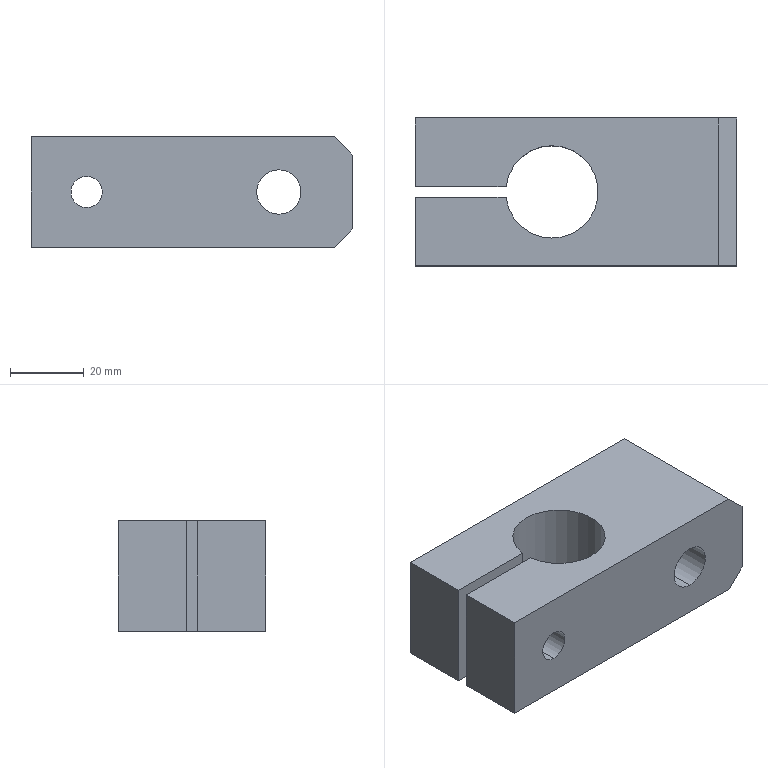Component | SolidWorks | DirectPressureVerticalSeal-1_VerticalSealMainArmFixingFrame-1 | 1 solid | 20 faces | box 87 x 40 x 30 mm | volume 79126 mm3 | plane 11 | cylinder 7 | cone 2 | commonest cylinder face diameters 11 x2 12 x2 8.5 x2 25 x1
STEP:
#1=CARTESIAN_POINT('',(-20.502,9.63,11.191));
#2=VERTEX_POINT('',#1);
#3=CARTESIAN_POINT('',(-20.502,9.63,11.526));
#4=VERTEX_POINT('',#3);
#5=CARTESIAN_POINT('',(-20.502,9.63,11.358));
#6=DIRECTION('',(0.,1.,0.));
#7=DIRECTION('',(0.,0.,-1.));
#8=AXIS2_PLACEMENT_3D('',#5,#6,#7);
#9=CIRCLE('',#8,0.1673);
#10=EDGE_CURVE('',#2,#4,#9,.T.);
#11=ORIENTED_EDGE('',*,*,#10,.F.);
#12=CARTESIAN_POINT('',(-20.502,9.66,11.16));
#13=VERTEX_POINT('',#12);
#14=CARTESIAN_POINT('',(-20.502,9.63,11.191));
#15=DIRECTION('',(0.,0.7071,-0.7071));
#16=VECTOR('',#15,39.37);
#17=LINE('',#14,#16);
#18=EDGE_CURVE('',#2,#13,#17,.T.);
#19=ORIENTED_EDGE('',*,*,#18,.T.);
#20=CARTESIAN_POINT('',(-20.502,9.66,11.556));
#21=VERTEX_POINT('',#20);
#22=CARTESIAN_POINT('',(-20.502,9.66,11.358));
#23=DIRECTION('',(-0.,-1.,0.));
#24=DIRECTION('',(1.,0.,0.));
#25=AXIS2_PLACEMENT_3D('',#22,#23,#24);
#26=CIRCLE('',#25,0.1978);
#27=EDGE_CURVE('',#21,#13,#26,.T.);
#28=ORIENTED_EDGE('',*,*,#27,.F.);
#29=CARTESIAN_POINT('',(-20.502,9.63,11.526));
#30=DIRECTION('',(0.,0.7071,0.7071));
#31=VECTOR('',#30,39.37);
#32=LINE('',#29,#31);
#33=EDGE_CURVE('',#4,#21,#32,.T.);
#34=ORIENTED_EDGE('',*,*,#33,.F.);
#35=EDGE_LOOP('',(#11,#19,#28,#34));
#36=FACE_OUTER_BOUND('',#35,.T.);
#37=CARTESIAN_POINT('',(-20.502,9.63,11.358));
#38=DIRECTION('',(0.,1.,0.));
#39=DIRECTION('',(0.,0.,1.));
#40=AXIS2_PLACEMENT_3D('',#37,#38,#39);
#41=CONICAL_SURFACE('',#40,0.1673,0.7854);
#42=ADVANCED_FACE('',(#36),#41,.F.);
#43=CARTESIAN_POINT('',(-20.502,10.507,11.575));
#44=VERTEX_POINT('',#43);
#45=CARTESIAN_POINT('',(-20.502,10.507,11.142));
#46=VERTEX_POINT('',#45);
#47=CARTESIAN_POINT('',(-20.502,10.507,11.358));
#48=DIRECTION('',(0.,-1.,0.));
#49=DIRECTION('',(0.,0.,-1.));
#50=AXIS2_PLACEMENT_3D('',#47,#48,#49);
#51=CIRCLE('',#50,0.2165);
#52=EDGE_CURVE('',#44,#46,#51,.T.);
#53=ORIENTED_EDGE('',*,*,#52,.F.);
#54=CARTESIAN_POINT('',(-20.502,9.778,11.575));
#55=VERTEX_POINT('',#54);
#56=CARTESIAN_POINT('',(-20.502,9.778,11.575));
#57=DIRECTION('',(0.,-1.,0.));
#58=VECTOR('',#57,39.37);
#59=LINE('',#56,#58);
#60=EDGE_CURVE('',#44,#55,#59,.T.);
#61=ORIENTED_EDGE('',*,*,#60,.T.);
#62=CARTESIAN_POINT('',(-20.502,9.778,11.142));
#63=VERTEX_POINT('',#62);
#64=CARTESIAN_POINT('',(-20.502,9.778,11.358));
#65=DIRECTION('',(0.,-1.,0.));
#66=DIRECTION('',(0.,0.,-1.));
#67=AXIS2_PLACEMENT_3D('',#64,#65,#66);
#68=CIRCLE('',#67,0.2165);
#69=EDGE_CURVE('',#55,#63,#68,.T.);
#70=ORIENTED_EDGE('',*,*,#69,.T.);
#71=CARTESIAN_POINT('',(-20.502,9.778,11.142));
#72=DIRECTION('',(0.,-1.,0.));
#73=VECTOR('',#72,39.37);
#74=LINE('',#71,#73);
#75=EDGE_CURVE('',#46,#63,#74,.T.);
#76=ORIENTED_EDGE('',*,*,#75,.F.);
#77=EDGE_LOOP('',(#53,#61,#70,#76));
#78=FACE_OUTER_BOUND('',#77,.T.);
#79=CARTESIAN_POINT('',(-20.502,9.778,11.358));
#80=DIRECTION('',(0.,-1.,0.));
#81=DIRECTION('',(0.,0.,-1.));
#82=AXIS2_PLACEMENT_3D('',#79,#80,#81);
#83=CYLINDRICAL_SURFACE('',#82,0.2165);
#84=ADVANCED_FACE('',(#78),#83,.F.);
#85=CARTESIAN_POINT('',(-18.455,10.507,11.594));
#86=VERTEX_POINT('',#85);
#87=CARTESIAN_POINT('',(-18.455,10.507,11.122));
#88=VERTEX_POINT('',#87);
#89=CARTESIAN_POINT('',(-18.455,10.507,11.358));
#90=DIRECTION('',(0.,-1.,0.));
#91=DIRECTION('',(0.,0.,-1.));
#92=AXIS2_PLACEMENT_3D('',#89,#90,#91);
#93=CIRCLE('',#92,0.2362);
#94=EDGE_CURVE('',#86,#88,#93,.T.);
#95=ORIENTED_EDGE('',*,*,#94,.F.);
#96=CARTESIAN_POINT('',(-18.455,8.932,11.594));
#97=VERTEX_POINT('',#96);
#98=CARTESIAN_POINT('',(-18.455,8.932,11.594));
#99=DIRECTION('',(0.,-1.,0.));
#100=VECTOR('',#99,39.37);
#101=LINE('',#98,#100);
#102=EDGE_CURVE('',#86,#97,#101,.T.);
#103=ORIENTED_EDGE('',*,*,#102,.T.);
#104=CARTESIAN_POINT('',(-18.455,8.932,11.122));
#105=VERTEX_POINT('',#104);
#106=CARTESIAN_POINT('',(-18.455,8.932,11.358));
#107=DIRECTION('',(0.,-1.,0.));
#108=DIRECTION('',(0.,0.,-1.));
#109=AXIS2_PLACEMENT_3D('',#106,#107,#108);
#110=CIRCLE('',#109,0.2362);
#111=EDGE_CURVE('',#97,#105,#110,.T.);
#112=ORIENTED_EDGE('',*,*,#111,.T.);
#113=CARTESIAN_POINT('',(-18.455,8.932,11.122));
#114=DIRECTION('',(0.,-1.,0.));
#115=VECTOR('',#114,39.37);
#116=LINE('',#113,#115);
#117=EDGE_CURVE('',#88,#105,#116,.T.);
#118=ORIENTED_EDGE('',*,*,#117,.F.);
#119=EDGE_LOOP('',(#95,#103,#112,#118));
#120=FACE_OUTER_BOUND('',#119,.T.);
#121=CARTESIAN_POINT('',(-18.455,8.932,11.358));
#122=DIRECTION('',(0.,-1.,0.));
#123=DIRECTION('',(0.,0.,-1.));
#124=AXIS2_PLACEMENT_3D('',#121,#122,#123);
#125=CYLINDRICAL_SURFACE('',#124,0.2362);
#126=ADVANCED_FACE('',(#120),#125,.F.);
#127=CARTESIAN_POINT('',(-20.502,8.932,11.191));
#128=VERTEX_POINT('',#127);
#129=CARTESIAN_POINT('',(-20.502,8.932,11.526));
#130=VERTEX_POINT('',#129);
#131=CARTESIAN_POINT('',(-20.502,8.932,11.358));
#132=DIRECTION('',(0.,1.,0.));
#133=DIRECTION('',(0.,0.,1.));
#134=AXIS2_PLACEMENT_3D('',#131,#132,#133);
#135=CIRCLE('',#134,0.1673);
#136=EDGE_CURVE('',#128,#130,#135,.T.);
#137=ORIENTED_EDGE('',*,*,#136,.F.);
#138=CARTESIAN_POINT('',(-20.502,9.66,11.191));
#139=DIRECTION('',(0.,1.,0.));
#140=VECTOR('',#139,39.37);
#141=LINE('',#138,#140);
#142=EDGE_CURVE('',#128,#2,#141,.T.);
#143=ORIENTED_EDGE('',*,*,#142,.T.);
#144=ORIENTED_EDGE('',*,*,#10,.T.);
#145=CARTESIAN_POINT('',(-20.502,9.66,11.526));
#146=DIRECTION('',(0.,1.,0.));
#147=VECTOR('',#146,39.37);
#148=LINE('',#145,#147);
#149=EDGE_CURVE('',#130,#4,#148,.T.);
#150=ORIENTED_EDGE('',*,*,#149,.F.);
#151=EDGE_LOOP('',(#137,#143,#144,#150));
#152=FACE_OUTER_BOUND('',#151,.T.);
#153=CARTESIAN_POINT('',(-20.502,9.66,11.358));
#154=DIRECTION('',(0.,1.,0.));
#155=DIRECTION('',(0.,0.,1.));
#156=AXIS2_PLACEMENT_3D('',#153,#154,#155);
#157=CYLINDRICAL_SURFACE('',#156,0.1673);
#158=ADVANCED_FACE('',(#152),#157,.F.);
#159=CARTESIAN_POINT('',(-21.092,9.66,11.949));
#160=VERTEX_POINT('',#159);
#161=CARTESIAN_POINT('',(-21.092,9.66,10.768));
#162=VERTEX_POINT('',#161);
#163=CARTESIAN_POINT('',(-21.092,9.66,11.949));
#164=DIRECTION('',(0.,0.,-1.));
#165=VECTOR('',#164,39.37);
#166=LINE('',#163,#165);
#167=EDGE_CURVE('',#160,#162,#166,.T.);
#168=ORIENTED_EDGE('',*,*,#167,.T.);
#169=CARTESIAN_POINT('',(-21.092,8.932,10.768));
#170=VERTEX_POINT('',#169);
#171=CARTESIAN_POINT('',(-21.092,10.507,10.768));
#172=DIRECTION('',(0.,-1.,0.));
#173=VECTOR('',#172,39.37);
#174=LINE('',#171,#173);
#175=EDGE_CURVE('',#162,#170,#174,.T.);
#176=ORIENTED_EDGE('',*,*,#175,.T.);
#177=CARTESIAN_POINT('',(-21.092,8.932,11.949));
#178=VERTEX_POINT('',#177);
#179=CARTESIAN_POINT('',(-21.092,8.932,10.768));
#180=DIRECTION('',(0.,0.,1.));
#181=VECTOR('',#180,39.37);
#182=LINE('',#179,#181);
#183=EDGE_CURVE('',#170,#178,#182,.T.);
#184=ORIENTED_EDGE('',*,*,#183,.T.);
#185=CARTESIAN_POINT('',(-21.092,10.507,11.949));
#186=DIRECTION('',(0.,-1.,0.));
#187=VECTOR('',#186,39.37);
#188=LINE('',#185,#187);
#189=EDGE_CURVE('',#160,#178,#188,.T.);
#190=ORIENTED_EDGE('',*,*,#189,.F.);
#191=EDGE_LOOP('',(#168,#176,#184,#190));
#192=FACE_OUTER_BOUND('',#191,.T.);
#193=CARTESIAN_POINT('',(-21.092,10.507,10.768));
#194=DIRECTION('',(-1.,0.,0.));
#195=DIRECTION('',(0.,0.,1.));
#196=AXIS2_PLACEMENT_3D('',#193,#194,#195);
#197=PLANE('',#196);
#198=ADVANCED_FACE('',(#192),#197,.T.);
#199=CARTESIAN_POINT('',(-17.667,8.932,10.965));
#200=VERTEX_POINT('',#199);
#201=CARTESIAN_POINT('',(-17.667,8.932,11.752));
#202=VERTEX_POINT('',#201);
#203=CARTESIAN_POINT('',(-17.667,8.932,10.768));
#204=DIRECTION('',(0.,0.,1.));
#205=VECTOR('',#204,39.37);
#206=LINE('',#203,#205);
#207=EDGE_CURVE('',#200,#202,#206,.T.);
#208=ORIENTED_EDGE('',*,*,#207,.F.);
#209=CARTESIAN_POINT('',(-17.667,10.507,10.965));
#210=VERTEX_POINT('',#209);
#211=CARTESIAN_POINT('',(-17.667,10.507,10.965));
#212=DIRECTION('',(0.,1.,0.));
#213=VECTOR('',#212,39.37);
#214=LINE('',#211,#213);
#215=EDGE_CURVE('',#200,#210,#214,.T.);
#216=ORIENTED_EDGE('',*,*,#215,.T.);
#217=CARTESIAN_POINT('',(-17.667,10.507,11.752));
#218=VERTEX_POINT('',#217);
#219=CARTESIAN_POINT('',(-17.667,10.507,10.768));
#220=DIRECTION('',(0.,0.,1.));
#221=VECTOR('',#220,39.37);
#222=LINE('',#219,#221);
#223=EDGE_CURVE('',#210,#218,#222,.T.);
#224=ORIENTED_EDGE('',*,*,#223,.T.);
#225=CARTESIAN_POINT('',(-17.667,8.932,11.752));
#226=DIRECTION('',(0.,-1.,0.));
#227=VECTOR('',#226,39.37);
#228=LINE('',#225,#227);
#229=EDGE_CURVE('',#218,#202,#228,.T.);
#230=ORIENTED_EDGE('',*,*,#229,.T.);
#231=EDGE_LOOP('',(#208,#216,#224,#230));
#232=FACE_OUTER_BOUND('',#231,.T.);
#233=CARTESIAN_POINT('',(-17.667,8.932,10.768));
#234=DIRECTION('',(1.,0.,0.));
#235=DIRECTION('',(0.,0.,-1.));
#236=AXIS2_PLACEMENT_3D('',#233,#234,#235);
#237=PLANE('',#236);
#238=ADVANCED_FACE('',(#232),#237,.T.);
#239=CARTESIAN_POINT('',(-18.455,8.932,11.358));
#240=DIRECTION('',(0.,-1.,0.));
#241=DIRECTION('',(0.,0.,-1.));
#242=AXIS2_PLACEMENT_3D('',#239,#240,#241);
#243=CIRCLE('',#242,0.2362);
#244=EDGE_CURVE('',#105,#97,#243,.T.);
#245=ORIENTED_EDGE('',*,*,#244,.F.);
#246=ORIENTED_EDGE('',*,*,#111,.F.);
#247=EDGE_LOOP('',(#245,#246));
#248=FACE_BOUND('',#247,.T.);
#249=CARTESIAN_POINT('',(-20.502,8.932,11.358));
#250=DIRECTION('',(0.,1.,0.));
#251=DIRECTION('',(0.,0.,1.));
#252=AXIS2_PLACEMENT_3D('',#249,#250,#251);
#253=CIRCLE('',#252,0.1673);
#254=EDGE_CURVE('',#130,#128,#253,.T.);
#255=ORIENTED_EDGE('',*,*,#254,.T.);
#256=ORIENTED_EDGE('',*,*,#136,.T.);
#257=EDGE_LOOP('',(#255,#256));
#258=FACE_BOUND('',#257,.T.);
#259=CARTESIAN_POINT('',(-17.864,8.932,10.768));
#260=VERTEX_POINT('',#259);
#261=CARTESIAN_POINT('',(-21.092,8.932,10.768));
#262=DIRECTION('',(1.,0.,0.));
#263=VECTOR('',#262,39.37);
#264=LINE('',#261,#263);
#265=EDGE_CURVE('',#170,#260,#264,.T.);
#266=ORIENTED_EDGE('',*,*,#265,.T.);
#267=CARTESIAN_POINT('',(-19.478,8.932,9.154));
#268=DIRECTION('',(0.7071,0.,0.7071));
#269=VECTOR('',#268,39.37);
#270=LINE('',#267,#269);
#271=EDGE_CURVE('',#260,#200,#270,.T.);
#272=ORIENTED_EDGE('',*,*,#271,.T.);
#273=ORIENTED_EDGE('',*,*,#207,.T.);
#274=CARTESIAN_POINT('',(-17.864,8.932,11.949));
#275=VERTEX_POINT('',#274);
#276=CARTESIAN_POINT('',(-18.888,8.932,12.972));
#277=DIRECTION('',(-0.7071,0.,0.7071));
#278=VECTOR('',#277,39.37);
#279=LINE('',#276,#278);
#280=EDGE_CURVE('',#202,#275,#279,.T.);
#281=ORIENTED_EDGE('',*,*,#280,.T.);
#282=CARTESIAN_POINT('',(-21.092,8.932,11.949));
#283=DIRECTION('',(1.,0.,0.));
#284=VECTOR('',#283,39.37);
#285=LINE('',#282,#284);
#286=EDGE_CURVE('',#178,#275,#285,.T.);
#287=ORIENTED_EDGE('',*,*,#286,.F.);
#288=ORIENTED_EDGE('',*,*,#183,.F.);
#289=EDGE_LOOP('',(#266,#272,#273,#281,#287,#288));
#290=FACE_OUTER_BOUND('',#289,.T.);
#291=CARTESIAN_POINT('',(-21.092,8.932,10.768));
#292=DIRECTION('',(0.,-1.,0.));
#293=DIRECTION('',(0.,0.,-1.));
#294=AXIS2_PLACEMENT_3D('',#291,#292,#293);
#295=PLANE('',#294);
#296=ADVANCED_FACE('',(#248,#258,#290),#295,.T.);
#297=CARTESIAN_POINT('',(-21.092,9.778,11.949));
#298=VERTEX_POINT('',#297);
#299=CARTESIAN_POINT('',(-21.092,9.778,10.768));
#300=VERTEX_POINT('',#299);
#301=CARTESIAN_POINT('',(-21.092,9.778,11.949));
#302=DIRECTION('',(0.,0.,-1.));
#303=VECTOR('',#302,39.37);
#304=LINE('',#301,#303);
#305=EDGE_CURVE('',#298,#300,#304,.T.);
#306=ORIENTED_EDGE('',*,*,#305,.F.);
#307=CARTESIAN_POINT('',(-21.092,10.507,11.949));
#308=VERTEX_POINT('',#307);
#309=CARTESIAN_POINT('',(-21.092,10.507,11.949));
#310=DIRECTION('',(0.,-1.,0.));
#311=VECTOR('',#310,39.37);
#312=LINE('',#309,#311);
#313=EDGE_CURVE('',#308,#298,#312,.T.);
#314=ORIENTED_EDGE('',*,*,#313,.F.);
#315=CARTESIAN_POINT('',(-21.092,10.507,10.768));
#316=VERTEX_POINT('',#315);
#317=CARTESIAN_POINT('',(-21.092,10.507,10.768));
#318=DIRECTION('',(0.,0.,1.));
#319=VECTOR('',#318,39.37);
#320=LINE('',#317,#319);
#321=EDGE_CURVE('',#316,#308,#320,.T.);
#322=ORIENTED_EDGE('',*,*,#321,.F.);
#323=CARTESIAN_POINT('',(-21.092,10.507,10.768));
#324=DIRECTION('',(0.,-1.,0.));
#325=VECTOR('',#324,39.37);
#326=LINE('',#323,#325);
#327=EDGE_CURVE('',#316,#300,#326,.T.);
#328=ORIENTED_EDGE('',*,*,#327,.T.);
#329=EDGE_LOOP('',(#306,#314,#322,#328));
#330=FACE_OUTER_BOUND('',#329,.T.);
#331=CARTESIAN_POINT('',(-21.092,10.507,10.768));
#332=DIRECTION('',(-1.,0.,0.));
#333=DIRECTION('',(0.,0.,1.));
#334=AXIS2_PLACEMENT_3D('',#331,#332,#333);
#335=PLANE('',#334);
#336=ADVANCED_FACE('',(#330),#335,.T.);
#337=CARTESIAN_POINT('',(-20.502,10.507,11.358));
#338=DIRECTION('',(0.,-1.,0.));
#339=DIRECTION('',(0.,0.,-1.));
#340=AXIS2_PLACEMENT_3D('',#337,#338,#339);
#341=CIRCLE('',#340,0.2165);
#342=EDGE_CURVE('',#46,#44,#341,.T.);
#343=ORIENTED_EDGE('',*,*,#342,.T.);
#344=ORIENTED_EDGE('',*,*,#52,.T.);
#345=EDGE_LOOP('',(#343,#344));
#346=FACE_BOUND('',#345,.T.);
#347=CARTESIAN_POINT('',(-18.455,10.507,11.358));
#348=DIRECTION('',(0.,-1.,0.));
#349=DIRECTION('',(0.,0.,-1.));
#350=AXIS2_PLACEMENT_3D('',#347,#348,#349);
#351=CIRCLE('',#350,0.2362);
#352=EDGE_CURVE('',#88,#86,#351,.T.);
#353=ORIENTED_EDGE('',*,*,#352,.T.);
#354=ORIENTED_EDGE('',*,*,#94,.T.);
#355=EDGE_LOOP('',(#353,#354));
#356=FACE_BOUND('',#355,.T.);
#357=ORIENTED_EDGE('',*,*,#223,.F.);
#358=CARTESIAN_POINT('',(-17.864,10.507,10.768));
#359=VERTEX_POINT('',#358);
#360=CARTESIAN_POINT('',(-17.766,10.507,10.866));
#361=DIRECTION('',(-0.7071,0.,-0.7071));
#362=VECTOR('',#361,39.37);
#363=LINE('',#360,#362);
#364=EDGE_CURVE('',#210,#359,#363,.T.);
#365=ORIENTED_EDGE('',*,*,#364,.T.);
#366=CARTESIAN_POINT('',(-17.667,10.507,10.768));
#367=DIRECTION('',(-1.,0.,0.));
#368=VECTOR('',#367,39.37);
#369=LINE('',#366,#368);
#370=EDGE_CURVE('',#359,#316,#369,.T.);
#371=ORIENTED_EDGE('',*,*,#370,.T.);
#372=ORIENTED_EDGE('',*,*,#321,.T.);
#373=CARTESIAN_POINT('',(-17.864,10.507,11.949));
#374=VERTEX_POINT('',#373);
#375=CARTESIAN_POINT('',(-17.667,10.507,11.949));
#376=DIRECTION('',(-1.,0.,0.));
#377=VECTOR('',#376,39.37);
#378=LINE('',#375,#377);
#379=EDGE_CURVE('',#374,#308,#378,.T.);
#380=ORIENTED_EDGE('',*,*,#379,.F.);
#381=CARTESIAN_POINT('',(-17.175,10.507,11.26));
#382=DIRECTION('',(0.7071,0.,-0.7071));
#383=VECTOR('',#382,39.37);
#384=LINE('',#381,#383);
#385=EDGE_CURVE('',#374,#218,#384,.T.);
#386=ORIENTED_EDGE('',*,*,#385,.T.);
#387=EDGE_LOOP('',(#357,#365,#371,#372,#380,#386));
#388=FACE_OUTER_BOUND('',#387,.T.);
#389=CARTESIAN_POINT('',(-17.667,10.507,10.768));
#390=DIRECTION('',(0.,1.,0.));
#391=DIRECTION('',(0.,0.,1.));
#392=AXIS2_PLACEMENT_3D('',#389,#390,#391);
#393=PLANE('',#392);
#394=ADVANCED_FACE('',(#346,#356,#388),#393,.T.);
#395=ORIENTED_EDGE('',*,*,#370,.F.);
#396=CARTESIAN_POINT('',(-17.864,8.932,10.768));
#397=DIRECTION('',(0.,-1.,0.));
#398=VECTOR('',#397,39.37);
#399=LINE('',#396,#398);
#400=EDGE_CURVE('',#359,#260,#399,.T.);
#401=ORIENTED_EDGE('',*,*,#400,.T.);
#402=ORIENTED_EDGE('',*,*,#265,.F.);
#403=ORIENTED_EDGE('',*,*,#175,.F.);
#404=CARTESIAN_POINT('',(-20.124,9.66,10.768));
#405=VERTEX_POINT('',#404);
#406=CARTESIAN_POINT('',(-20.124,9.66,10.768));
#407=DIRECTION('',(-1.,0.,0.));
#408=VECTOR('',#407,39.37);
#409=LINE('',#406,#408);
#410=EDGE_CURVE('',#405,#162,#409,.T.);
#411=ORIENTED_EDGE('',*,*,#410,.F.);
#412=CARTESIAN_POINT('',(-20.124,9.778,10.768));
#413=VERTEX_POINT('',#412);
#414=CARTESIAN_POINT('',(-19.636,9.719,10.768));
#415=DIRECTION('',(0.,0.,-1.));
#416=DIRECTION('',(-1.,0.,0.));
#417=AXIS2_PLACEMENT_3D('',#414,#415,#416);
#418=CIRCLE('',#417,0.4921);
#419=EDGE_CURVE('',#413,#405,#418,.T.);
#420=ORIENTED_EDGE('',*,*,#419,.F.);
#421=CARTESIAN_POINT('',(-21.092,9.778,10.768));
#422=DIRECTION('',(1.,0.,0.));
#423=VECTOR('',#422,39.37);
#424=LINE('',#421,#423);
#425=EDGE_CURVE('',#300,#413,#424,.T.);
#426=ORIENTED_EDGE('',*,*,#425,.F.);
#427=ORIENTED_EDGE('',*,*,#327,.F.);
#428=EDGE_LOOP('',(#395,#401,#402,#403,#411,#420,#426,#427));
#429=FACE_OUTER_BOUND('',#428,.T.);
#430=CARTESIAN_POINT('',(-19.38,9.719,10.768));
#431=DIRECTION('',(0.,0.,1.));
#432=DIRECTION('',(1.,0.,0.));
#433=AXIS2_PLACEMENT_3D('',#430,#431,#432);
#434=PLANE('',#433);
#435=ADVANCED_FACE('',(#429),#434,.F.);
#436=ORIENTED_EDGE('',*,*,#286,.T.);
#437=CARTESIAN_POINT('',(-17.864,9.719,11.949));
#438=DIRECTION('',(0.,1.,0.));
#439=VECTOR('',#438,39.37);
#440=LINE('',#437,#439);
#441=EDGE_CURVE('',#275,#374,#440,.T.);
#442=ORIENTED_EDGE('',*,*,#441,.T.);
#443=ORIENTED_EDGE('',*,*,#379,.T.);
#444=ORIENTED_EDGE('',*,*,#313,.T.);
#445=CARTESIAN_POINT('',(-20.124,9.778,11.949));
#446=VERTEX_POINT('',#445);
#447=CARTESIAN_POINT('',(-21.092,9.778,11.949));
#448=DIRECTION('',(1.,0.,0.));
#449=VECTOR('',#448,39.37);
#450=LINE('',#447,#449);
#451=EDGE_CURVE('',#298,#446,#450,.T.);
#452=ORIENTED_EDGE('',*,*,#451,.T.);
#453=CARTESIAN_POINT('',(-20.124,9.66,11.949));
#454=VERTEX_POINT('',#453);
#455=CARTESIAN_POINT('',(-19.636,9.719,11.949));
#456=DIRECTION('',(0.,0.,-1.));
#457=DIRECTION('',(-1.,0.,0.));
#458=AXIS2_PLACEMENT_3D('',#455,#456,#457);
#459=CIRCLE('',#458,0.4921);
#460=EDGE_CURVE('',#446,#454,#459,.T.);
#461=ORIENTED_EDGE('',*,*,#460,.T.);
#462=CARTESIAN_POINT('',(-20.124,9.66,11.949));
#463=DIRECTION('',(-1.,0.,0.));
#464=VECTOR('',#463,39.37);
#465=LINE('',#462,#464);
#466=EDGE_CURVE('',#454,#160,#465,.T.);
#467=ORIENTED_EDGE('',*,*,#466,.T.);
#468=ORIENTED_EDGE('',*,*,#189,.T.);
#469=EDGE_LOOP('',(#436,#442,#443,#444,#452,#461,#467,#468));
#470=FACE_OUTER_BOUND('',#469,.T.);
#471=CARTESIAN_POINT('',(-19.38,9.719,11.949));
#472=DIRECTION('',(0.,0.,1.));
#473=DIRECTION('',(1.,0.,0.));
#474=AXIS2_PLACEMENT_3D('',#471,#472,#473);
#475=PLANE('',#474);
#476=ADVANCED_FACE('',(#470),#475,.T.);
#477=ORIENTED_EDGE('',*,*,#27,.T.);
#478=CARTESIAN_POINT('',(-20.502,9.66,11.358));
#479=DIRECTION('',(-0.,-1.,0.));
#480=DIRECTION('',(1.,0.,0.));
#481=AXIS2_PLACEMENT_3D('',#478,#479,#480);
#482=CIRCLE('',#481,0.1978);
#483=EDGE_CURVE('',#13,#21,#482,.T.);
#484=ORIENTED_EDGE('',*,*,#483,.T.);
#485=EDGE_LOOP('',(#477,#484));
#486=FACE_BOUND('',#485,.T.);
#487=ORIENTED_EDGE('',*,*,#410,.T.);
#488=ORIENTED_EDGE('',*,*,#167,.F.);
#489=ORIENTED_EDGE('',*,*,#466,.F.);
#490=CARTESIAN_POINT('',(-20.124,9.66,11.949));
#491=DIRECTION('',(0.,0.,-1.));
#492=VECTOR('',#491,39.37);
#493=LINE('',#490,#492);
#494=EDGE_CURVE('',#454,#405,#493,.T.);
#495=ORIENTED_EDGE('',*,*,#494,.T.);
#496=EDGE_LOOP('',(#487,#488,#489,#495));
#497=FACE_OUTER_BOUND('',#496,.T.);
#498=CARTESIAN_POINT('',(-20.124,9.66,11.949));
#499=DIRECTION('',(-0.,-1.,0.));
#500=DIRECTION('',(1.,-0.,0.));
#501=AXIS2_PLACEMENT_3D('',#498,#499,#500);
#502=PLANE('',#501);
#503=ADVANCED_FACE('',(#486,#497),#502,.F.);
#504=CARTESIAN_POINT('',(-20.502,9.778,11.358));
#505=DIRECTION('',(0.,-1.,0.));
#506=DIRECTION('',(0.,0.,-1.));
#507=AXIS2_PLACEMENT_3D('',#504,#505,#506);
#508=CIRCLE('',#507,0.2165);
#509=EDGE_CURVE('',#63,#55,#508,.T.);
#510=ORIENTED_EDGE('',*,*,#509,.F.);
#511=ORIENTED_EDGE('',*,*,#69,.F.);
#512=EDGE_LOOP('',(#510,#511));
#513=FACE_BOUND('',#512,.T.);
#514=ORIENTED_EDGE('',*,*,#425,.T.);
#515=CARTESIAN_POINT('',(-20.124,9.778,11.949));
#516=DIRECTION('',(0.,0.,-1.));
#517=VECTOR('',#516,39.37);
#518=LINE('',#515,#517);
#519=EDGE_CURVE('',#446,#413,#518,.T.);
#520=ORIENTED_EDGE('',*,*,#519,.F.);
#521=ORIENTED_EDGE('',*,*,#451,.F.);
#522=ORIENTED_EDGE('',*,*,#305,.T.);
#523=EDGE_LOOP('',(#514,#520,#521,#522));
#524=FACE_OUTER_BOUND('',#523,.T.);
#525=CARTESIAN_POINT('',(-21.092,9.778,11.949));
#526=DIRECTION('',(-0.,1.,0.));
#527=DIRECTION('',(-1.,-0.,0.));
#528=AXIS2_PLACEMENT_3D('',#525,#526,#527);
#529=PLANE('',#528);
#530=ADVANCED_FACE('',(#513,#524),#529,.F.);
#531=ORIENTED_EDGE('',*,*,#460,.F.);
#532=ORIENTED_EDGE('',*,*,#519,.T.);
#533=ORIENTED_EDGE('',*,*,#419,.T.);
#534=ORIENTED_EDGE('',*,*,#494,.F.);
#535=EDGE_LOOP('',(#531,#532,#533,#534));
#536=FACE_OUTER_BOUND('',#535,.T.);
#537=CARTESIAN_POINT('',(-19.636,9.719,11.949));
#538=DIRECTION('',(0.,0.,-1.));
#539=DIRECTION('',(-1.,0.,0.));
#540=AXIS2_PLACEMENT_3D('',#537,#538,#539);
#541=CYLINDRICAL_SURFACE('',#540,0.4921);
#542=ADVANCED_FACE('',(#536),#541,.F.);
#543=ORIENTED_EDGE('',*,*,#142,.F.);
#544=ORIENTED_EDGE('',*,*,#254,.F.);
#545=ORIENTED_EDGE('',*,*,#149,.T.);
#546=CARTESIAN_POINT('',(-20.502,9.63,11.358));
#547=DIRECTION('',(0.,1.,0.));
#548=DIRECTION('',(0.,0.,-1.));
#549=AXIS2_PLACEMENT_3D('',#546,#547,#548);
#550=CIRCLE('',#549,0.1673);
#551=EDGE_CURVE('',#4,#2,#550,.T.);
#552=ORIENTED_EDGE('',*,*,#551,.T.);
#553=EDGE_LOOP('',(#543,#544,#545,#552));
#554=FACE_OUTER_BOUND('',#553,.T.);
#555=CARTESIAN_POINT('',(-20.502,9.66,11.358));
#556=DIRECTION('',(0.,1.,0.));
#557=DIRECTION('',(0.,0.,1.));
#558=AXIS2_PLACEMENT_3D('',#555,#556,#557);
#559=CYLINDRICAL_SURFACE('',#558,0.1673);
#560=ADVANCED_FACE('',(#554),#559,.F.);
#561=ORIENTED_EDGE('',*,*,#102,.F.);
#562=ORIENTED_EDGE('',*,*,#352,.F.);
#563=ORIENTED_EDGE('',*,*,#117,.T.);
#564=ORIENTED_EDGE('',*,*,#244,.T.);
#565=EDGE_LOOP('',(#561,#562,#563,#564));
#566=FACE_OUTER_BOUND('',#565,.T.);
#567=CARTESIAN_POINT('',(-18.455,8.932,11.358));
#568=DIRECTION('',(0.,-1.,0.));
#569=DIRECTION('',(0.,0.,-1.));
#570=AXIS2_PLACEMENT_3D('',#567,#568,#569);
#571=CYLINDRICAL_SURFACE('',#570,0.2362);
#572=ADVANCED_FACE('',(#566),#571,.F.);
#573=ORIENTED_EDGE('',*,*,#60,.F.);
#574=ORIENTED_EDGE('',*,*,#342,.F.);
#575=ORIENTED_EDGE('',*,*,#75,.T.);
#576=ORIENTED_EDGE('',*,*,#509,.T.);
#577=EDGE_LOOP('',(#573,#574,#575,#576));
#578=FACE_OUTER_BOUND('',#577,.T.);
#579=CARTESIAN_POINT('',(-20.502,9.778,11.358));
#580=DIRECTION('',(0.,-1.,0.));
#581=DIRECTION('',(0.,0.,-1.));
#582=AXIS2_PLACEMENT_3D('',#579,#580,#581);
#583=CYLINDRICAL_SURFACE('',#582,0.2165);
#584=ADVANCED_FACE('',(#578),#583,.F.);
#585=ORIENTED_EDGE('',*,*,#271,.F.);
#586=ORIENTED_EDGE('',*,*,#400,.F.);
#587=ORIENTED_EDGE('',*,*,#364,.F.);
#588=ORIENTED_EDGE('',*,*,#215,.F.);
#589=EDGE_LOOP('',(#585,#586,#587,#588));
#590=FACE_OUTER_BOUND('',#589,.T.);
#591=CARTESIAN_POINT('',(-17.667,8.932,10.965));
#592=DIRECTION('',(0.7071,0.,-0.7071));
#593=DIRECTION('',(0.,-1.,0.));
#594=AXIS2_PLACEMENT_3D('',#591,#592,#593);
#595=PLANE('',#594);
#596=ADVANCED_FACE('',(#590),#595,.T.);
#597=ORIENTED_EDGE('',*,*,#280,.F.);
#598=ORIENTED_EDGE('',*,*,#229,.F.);
#599=ORIENTED_EDGE('',*,*,#385,.F.);
#600=ORIENTED_EDGE('',*,*,#441,.F.);
#601=EDGE_LOOP('',(#597,#598,#599,#600));
#602=FACE_OUTER_BOUND('',#601,.T.);
#603=CARTESIAN_POINT('',(-17.864,9.719,11.949));
#604=DIRECTION('',(-0.7071,0.,-0.7071));
#605=DIRECTION('',(0.,1.,0.));
#606=AXIS2_PLACEMENT_3D('',#603,#604,#605);
#607=PLANE('',#606);
#608=ADVANCED_FACE('',(#602),#607,.F.);
#609=ORIENTED_EDGE('',*,*,#18,.F.);
#610=ORIENTED_EDGE('',*,*,#551,.F.);
#611=ORIENTED_EDGE('',*,*,#33,.T.);
#612=ORIENTED_EDGE('',*,*,#483,.F.);
#613=EDGE_LOOP('',(#609,#610,#611,#612));
#614=FACE_OUTER_BOUND('',#613,.T.);
#615=CARTESIAN_POINT('',(-20.502,9.63,11.358));
#616=DIRECTION('',(0.,1.,0.));
#617=DIRECTION('',(0.,0.,1.));
#618=AXIS2_PLACEMENT_3D('',#615,#616,#617);
#619=CONICAL_SURFACE('',#618,0.1673,0.7854);
#620=ADVANCED_FACE('',(#614),#619,.F.);
#621=CLOSED_SHELL('',(#42,#84,#126,#158,#198,#238,#296,#336,#394,#435,#476,#503,#530,#542,#560,#572,#584,#596,#608,#620));
#622=MANIFOLD_SOLID_BREP('',#621);
#623=CARTESIAN_POINT('',(0.,0.,0.));
#624=DIRECTION('',(0.,0.,1.));
#625=DIRECTION('',(1.,0.,0.));
#626=AXIS2_PLACEMENT_3D('',#623,#624,#625);
#627=(LENGTH_UNIT()NAMED_UNIT(*)SI_UNIT($,.METRE.));
#628=LENGTH_MEASURE_WITH_UNIT(LENGTH_MEASURE(0.0254),#627);
#629=DIMENSIONAL_EXPONENTS(1.,0.,0.,0.,0.,0.,0.);
#630=(CONVERSION_BASED_UNIT('',#628)LENGTH_UNIT()NAMED_UNIT(#629));
#631=UNCERTAINTY_MEASURE_WITH_UNIT(LENGTH_MEASURE(0.00001),#630,'','');
#632=(NAMED_UNIT(*)PLANE_ANGLE_UNIT()SI_UNIT($,.RADIAN.));
#633=(NAMED_UNIT(*)SI_UNIT($,.STERADIAN.)SOLID_ANGLE_UNIT());
#634=(GEOMETRIC_REPRESENTATION_CONTEXT(3)GLOBAL_UNCERTAINTY_ASSIGNED_CONTEXT((#631))GLOBAL_UNIT_ASSIGNED_CONTEXT((#630,#632,#633))REPRESENTATION_CONTEXT('',''));
#635=ADVANCED_BREP_SHAPE_REPRESENTATION('',(#622,#626),#634);
#636=COLOUR_RGB('',0.7922,0.8196,0.9333);
#637=FILL_AREA_STYLE_COLOUR('',#636);
#638=FILL_AREA_STYLE('',(#637));
#639=SURFACE_STYLE_FILL_AREA(#638);
#640=SURFACE_SIDE_STYLE('',(#639));
#641=SURFACE_STYLE_USAGE(.BOTH.,#640);
#642=PRESENTATION_STYLE_ASSIGNMENT((#641));
#643=STYLED_ITEM('',(#642),#622);
#644=PRESENTATION_LAYER_ASSIGNMENT('','',(#643));
#645=(LENGTH_UNIT()NAMED_UNIT(*)SI_UNIT($,.METRE.));
#646=LENGTH_MEASURE_WITH_UNIT(LENGTH_MEASURE(0.0254),#645);
#647=DIMENSIONAL_EXPONENTS(1.,0.,0.,0.,0.,0.,0.);
#648=(CONVERSION_BASED_UNIT('',#646)LENGTH_UNIT()NAMED_UNIT(#647));
#649=UNCERTAINTY_MEASURE_WITH_UNIT(LENGTH_MEASURE(0.00001),#648,'','');
#650=(NAMED_UNIT(*)PLANE_ANGLE_UNIT()SI_UNIT($,.RADIAN.));
#651=(NAMED_UNIT(*)SI_UNIT($,.STERADIAN.)SOLID_ANGLE_UNIT());
#652=(GEOMETRIC_REPRESENTATION_CONTEXT(3)GLOBAL_UNCERTAINTY_ASSIGNED_CONTEXT((#649))GLOBAL_UNIT_ASSIGNED_CONTEXT((#648,#650,#651))REPRESENTATION_CONTEXT('',''));
#653=MECHANICAL_DESIGN_GEOMETRIC_PRESENTATION_REPRESENTATION('',(#643),#652);